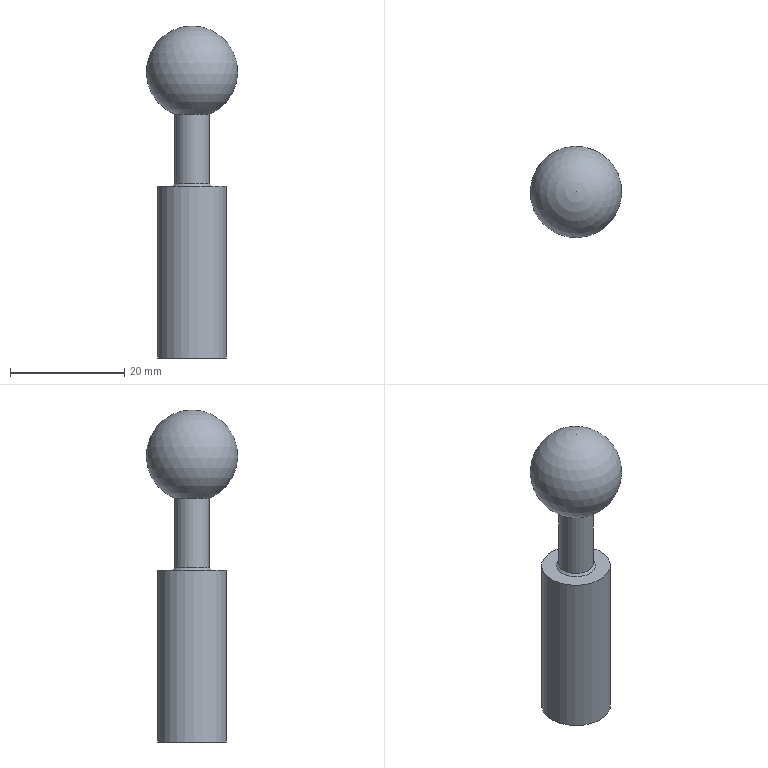Component | NX | GUIDE_POST | 1 solid | 6 faces | box 16 x 16 x 58 mm | volume 5887 mm3 | cylinder 2 | plane 2 | sphere 1 | cone 1 | commonest cylinder face diameters 6 x1 12 x1
STEP:
#1=CARTESIAN_POINT('',(0.,0.,0.));
#2=DIRECTION('',(0.,0.,1.));
#3=DIRECTION('',(1.,0.,0.));
#4=AXIS2_PLACEMENT_3D('',#1,#2,#3);
#5=CARTESIAN_POINT('',(-71.09,-2.544,40.4));
#6=VERTEX_POINT('',#5);
#7=CARTESIAN_POINT('',(-69.5,-0.,40.4));
#8=DIRECTION('',(0.,0.,1.));
#9=DIRECTION('',(-0.53,-0.848,0.));
#10=AXIS2_PLACEMENT_3D('',#7,#8,#9);
#11=CIRCLE('',#10,3.);
#12=CARTESIAN_POINT('',(-69.5,-0.,10.));
#13=DIRECTION('',(0.,0.,-1.));
#14=DIRECTION('',(-0.53,-0.848,0.));
#15=AXIS2_PLACEMENT_3D('',#12,#13,#14);
#16=CYLINDRICAL_SURFACE('',#15,3.);
#17=CARTESIAN_POINT('',(6.283,-30.4));
#18=DIRECTION('',(-1.,0.));
#19=VECTOR('',#18,1.);
#20=LINE('',#17,#19);
#21=(GEOMETRIC_REPRESENTATION_CONTEXT(2)PARAMETRIC_REPRESENTATION_CONTEXT()REPRESENTATION_CONTEXT('',''));
#22=DEFINITIONAL_REPRESENTATION('',(#20),#21);
#23=PCURVE('',#16,#22);
#24=CARTESIAN_POINT('',(-69.5,-0.,40.));
#25=DIRECTION('',(0.,0.,-1.));
#26=DIRECTION('',(-0.53,-0.848,0.));
#27=AXIS2_PLACEMENT_3D('',#24,#25,#26);
#28=CONICAL_SURFACE('',#27,3.4,0.7854);
#29=CARTESIAN_POINT('',(6.283,-0.4));
#30=DIRECTION('',(-1.,0.));
#31=VECTOR('',#30,1.);
#32=LINE('',#29,#31);
#33=(GEOMETRIC_REPRESENTATION_CONTEXT(2)PARAMETRIC_REPRESENTATION_CONTEXT()REPRESENTATION_CONTEXT('',''));
#34=DEFINITIONAL_REPRESENTATION('',(#32),#33);
#35=PCURVE('',#28,#34);
#36=SURFACE_CURVE('',#11,(#23,#35),.PCURVE_S1.);
#37=EDGE_CURVE('',#6,#6,#36,.T.);
#38=ORIENTED_EDGE('',*,*,#37,.T.);
#39=CARTESIAN_POINT('',(-71.09,-2.544,52.584));
#40=VERTEX_POINT('',#39);
#41=CARTESIAN_POINT('',(-71.09,-2.544,52.584));
#42=CARTESIAN_POINT('',(-71.09,-2.544,40.4));
#43=B_SPLINE_CURVE_WITH_KNOTS('',1,(#41,#42),.UNSPECIFIED.,.F.,.F.,(2,2),(-42.584,-30.4),.PIECEWISE_BEZIER_KNOTS.);
#44=CARTESIAN_POINT('',(0.,0.));
#45=DIRECTION('',(0.,1.));
#46=VECTOR('',#45,1.);
#47=LINE('',#44,#46);
#48=(GEOMETRIC_REPRESENTATION_CONTEXT(2)PARAMETRIC_REPRESENTATION_CONTEXT()REPRESENTATION_CONTEXT('',''));
#49=DEFINITIONAL_REPRESENTATION('',(#47),#48);
#50=PCURVE('',#16,#49);
#51=CARTESIAN_POINT('',(6.283,0.));
#52=DIRECTION('',(0.,1.));
#53=VECTOR('',#52,1.);
#54=LINE('',#51,#53);
#55=(GEOMETRIC_REPRESENTATION_CONTEXT(2)PARAMETRIC_REPRESENTATION_CONTEXT()REPRESENTATION_CONTEXT('',''));
#56=DEFINITIONAL_REPRESENTATION('',(#54),#55);
#57=PCURVE('',#16,#56);
#58=SEAM_CURVE('',#43,(#50,#57),.PCURVE_S1.);
#59=EDGE_CURVE('',#40,#6,#58,.T.);
#60=ORIENTED_EDGE('',*,*,#59,.F.);
#61=CARTESIAN_POINT('',(-67.91,2.544,52.584));
#62=VERTEX_POINT('',#61);
#63=CARTESIAN_POINT('',(-69.5,-0.,52.584));
#64=DIRECTION('',(0.,0.,-1.));
#65=DIRECTION('',(0.53,0.848,0.));
#66=AXIS2_PLACEMENT_3D('',#63,#64,#65);
#67=CIRCLE('',#66,3.);
#68=CARTESIAN_POINT('',(-3.142,-42.584));
#69=DIRECTION('',(1.,0.));
#70=VECTOR('',#69,1.);
#71=LINE('',#68,#70);
#72=(GEOMETRIC_REPRESENTATION_CONTEXT(2)PARAMETRIC_REPRESENTATION_CONTEXT()REPRESENTATION_CONTEXT('',''));
#73=DEFINITIONAL_REPRESENTATION('',(#71),#72);
#74=PCURVE('',#16,#73);
#75=CARTESIAN_POINT('',(-69.5,-0.,60.));
#76=DIRECTION('',(0.,0.,1.));
#77=DIRECTION('',(0.53,0.848,-0.));
#78=AXIS2_PLACEMENT_3D('',#75,#76,#77);
#79=SPHERICAL_SURFACE('',#78,8.);
#80=CARTESIAN_POINT('',(3.142,-1.186));
#81=CARTESIAN_POINT('',(3.094,-1.186));
#82=CARTESIAN_POINT('',(2.999,-1.186));
#83=CARTESIAN_POINT('',(2.856,-1.186));
#84=CARTESIAN_POINT('',(2.713,-1.186));
#85=CARTESIAN_POINT('',(2.57,-1.186));
#86=CARTESIAN_POINT('',(2.428,-1.186));
#87=CARTESIAN_POINT('',(2.285,-1.186));
#88=CARTESIAN_POINT('',(2.142,-1.186));
#89=CARTESIAN_POINT('',(1.999,-1.186));
#90=CARTESIAN_POINT('',(1.856,-1.186));
#91=CARTESIAN_POINT('',(1.714,-1.186));
#92=CARTESIAN_POINT('',(1.571,-1.186));
#93=CARTESIAN_POINT('',(1.428,-1.186));
#94=CARTESIAN_POINT('',(1.285,-1.186));
#95=CARTESIAN_POINT('',(1.142,-1.186));
#96=CARTESIAN_POINT('',(0.9996,-1.186));
#97=CARTESIAN_POINT('',(0.8568,-1.186));
#98=CARTESIAN_POINT('',(0.714,-1.186));
#99=CARTESIAN_POINT('',(0.5712,-1.186));
#100=CARTESIAN_POINT('',(0.4284,-1.186));
#101=CARTESIAN_POINT('',(0.2856,-1.186));
#102=CARTESIAN_POINT('',(0.1428,-1.186));
#103=CARTESIAN_POINT('',(0.0476,-1.186));
#104=CARTESIAN_POINT('',(0.,-1.186));
#105=B_SPLINE_CURVE_WITH_KNOTS('',3,(#80,#81,#82,#83,#84,#85,#86,#87,#88,#89,#90,#91,#92,#93,#94,#95,#96,#97,#98,#99,#100,#101,#102,#103,#104),.UNSPECIFIED.,.F.,.F.,(4,1,1,1,1,1,1,1,1,1,1,1,1,1,1,1,1,1,1,1,1,1,4),(3.142,3.284,3.427,3.57,3.713,3.856,3.998,4.141,4.284,4.427,4.57,4.712,4.855,4.998,5.141,5.284,5.426,5.569,5.712,5.855,5.998,6.14,6.283),.QUASI_UNIFORM_KNOTS.);
#106=(GEOMETRIC_REPRESENTATION_CONTEXT(2)PARAMETRIC_REPRESENTATION_CONTEXT()REPRESENTATION_CONTEXT('',''));
#107=DEFINITIONAL_REPRESENTATION('',(#105),#106);
#108=PCURVE('',#79,#107);
#109=SURFACE_CURVE('',#67,(#74,#108),.PCURVE_S1.);
#110=EDGE_CURVE('',#40,#62,#109,.T.);
#111=ORIENTED_EDGE('',*,*,#110,.T.);
#112=CARTESIAN_POINT('',(-69.5,-0.,52.584));
#113=DIRECTION('',(0.,0.,-1.));
#114=DIRECTION('',(0.53,0.848,0.));
#115=AXIS2_PLACEMENT_3D('',#112,#113,#114);
#116=CIRCLE('',#115,3.);
#117=CARTESIAN_POINT('',(3.142,-42.584));
#118=DIRECTION('',(1.,0.));
#119=VECTOR('',#118,1.);
#120=LINE('',#117,#119);
#121=(GEOMETRIC_REPRESENTATION_CONTEXT(2)PARAMETRIC_REPRESENTATION_CONTEXT()REPRESENTATION_CONTEXT('',''));
#122=DEFINITIONAL_REPRESENTATION('',(#120),#121);
#123=PCURVE('',#16,#122);
#124=CARTESIAN_POINT('',(6.283,-1.186));
#125=CARTESIAN_POINT('',(6.236,-1.186));
#126=CARTESIAN_POINT('',(6.14,-1.186));
#127=CARTESIAN_POINT('',(5.998,-1.186));
#128=CARTESIAN_POINT('',(5.855,-1.186));
#129=CARTESIAN_POINT('',(5.712,-1.186));
#130=CARTESIAN_POINT('',(5.569,-1.186));
#131=CARTESIAN_POINT('',(5.426,-1.186));
#132=CARTESIAN_POINT('',(5.284,-1.186));
#133=CARTESIAN_POINT('',(5.141,-1.186));
#134=CARTESIAN_POINT('',(4.998,-1.186));
#135=CARTESIAN_POINT('',(4.855,-1.186));
#136=CARTESIAN_POINT('',(4.712,-1.186));
#137=CARTESIAN_POINT('',(4.57,-1.186));
#138=CARTESIAN_POINT('',(4.427,-1.186));
#139=CARTESIAN_POINT('',(4.284,-1.186));
#140=CARTESIAN_POINT('',(4.141,-1.186));
#141=CARTESIAN_POINT('',(3.998,-1.186));
#142=CARTESIAN_POINT('',(3.856,-1.186));
#143=CARTESIAN_POINT('',(3.713,-1.186));
#144=CARTESIAN_POINT('',(3.57,-1.186));
#145=CARTESIAN_POINT('',(3.427,-1.186));
#146=CARTESIAN_POINT('',(3.284,-1.186));
#147=CARTESIAN_POINT('',(3.189,-1.186));
#148=CARTESIAN_POINT('',(3.142,-1.186));
#149=B_SPLINE_CURVE_WITH_KNOTS('',3,(#124,#125,#126,#127,#128,#129,#130,#131,#132,#133,#134,#135,#136,#137,#138,#139,#140,#141,#142,#143,#144,#145,#146,#147,#148),.UNSPECIFIED.,.F.,.F.,(4,1,1,1,1,1,1,1,1,1,1,1,1,1,1,1,1,1,1,1,1,1,4),(0.,0.1428,0.2856,0.4284,0.5712,0.714,0.8568,0.9996,1.142,1.285,1.428,1.571,1.714,1.856,1.999,2.142,2.285,2.428,2.57,2.713,2.856,2.999,3.142),.QUASI_UNIFORM_KNOTS.);
#150=(GEOMETRIC_REPRESENTATION_CONTEXT(2)PARAMETRIC_REPRESENTATION_CONTEXT()REPRESENTATION_CONTEXT('',''));
#151=DEFINITIONAL_REPRESENTATION('',(#149),#150);
#152=PCURVE('',#79,#151);
#153=SURFACE_CURVE('',#116,(#123,#152),.PCURVE_S1.);
#154=EDGE_CURVE('',#62,#40,#153,.T.);
#155=ORIENTED_EDGE('',*,*,#154,.T.);
#156=ORIENTED_EDGE('',*,*,#59,.T.);
#157=EDGE_LOOP('',(#38,#60,#111,#155,#156));
#158=FACE_BOUND('',#157,.T.);
#159=ADVANCED_FACE('',(#158),#16,.T.);
#160=CARTESIAN_POINT('',(-71.302,-2.883,40.));
#161=VERTEX_POINT('',#160);
#162=CARTESIAN_POINT('',(-69.5,-0.,40.));
#163=DIRECTION('',(0.,0.,-1.));
#164=DIRECTION('',(-0.53,-0.848,0.));
#165=AXIS2_PLACEMENT_3D('',#162,#163,#164);
#166=CIRCLE('',#165,3.4);
#167=CARTESIAN_POINT('',(-72.044,1.59,40.));
#168=DIRECTION('',(0.,0.,-1.));
#169=DIRECTION('',(-0.53,-0.848,0.));
#170=AXIS2_PLACEMENT_3D('',#167,#168,#169);
#171=PLANE('',#170);
#172=CARTESIAN_POINT('',(-0.,-3.));
#173=DIRECTION('',(1.,0.));
#174=AXIS2_PLACEMENT_2D('',#172,#173);
#175=CIRCLE('',#174,3.4);
#176=(GEOMETRIC_REPRESENTATION_CONTEXT(2)PARAMETRIC_REPRESENTATION_CONTEXT()REPRESENTATION_CONTEXT('',''));
#177=DEFINITIONAL_REPRESENTATION('',(#175),#176);
#178=PCURVE('',#171,#177);
#179=CARTESIAN_POINT('',(0.,0.));
#180=DIRECTION('',(1.,0.));
#181=VECTOR('',#180,1.);
#182=LINE('',#179,#181);
#183=(GEOMETRIC_REPRESENTATION_CONTEXT(2)PARAMETRIC_REPRESENTATION_CONTEXT()REPRESENTATION_CONTEXT('',''));
#184=DEFINITIONAL_REPRESENTATION('',(#182),#183);
#185=PCURVE('',#28,#184);
#186=SURFACE_CURVE('',#166,(#178,#185),.PCURVE_S1.);
#187=EDGE_CURVE('',#161,#161,#186,.T.);
#188=ORIENTED_EDGE('',*,*,#187,.T.);
#189=EDGE_LOOP('',(#188));
#190=FACE_BOUND('',#189,.T.);
#191=CARTESIAN_POINT('',(-72.68,-5.088,40.));
#192=VERTEX_POINT('',#191);
#193=CARTESIAN_POINT('',(-69.5,-0.,40.));
#194=DIRECTION('',(0.,0.,-1.));
#195=DIRECTION('',(-0.53,-0.848,0.));
#196=AXIS2_PLACEMENT_3D('',#193,#194,#195);
#197=CIRCLE('',#196,6.);
#198=CARTESIAN_POINT('',(-0.,-3.));
#199=DIRECTION('',(1.,0.));
#200=AXIS2_PLACEMENT_2D('',#198,#199);
#201=CIRCLE('',#200,6.);
#202=(GEOMETRIC_REPRESENTATION_CONTEXT(2)PARAMETRIC_REPRESENTATION_CONTEXT()REPRESENTATION_CONTEXT('',''));
#203=DEFINITIONAL_REPRESENTATION('',(#201),#202);
#204=PCURVE('',#171,#203);
#205=CARTESIAN_POINT('',(-69.5,-0.,10.));
#206=DIRECTION('',(0.,0.,-1.));
#207=DIRECTION('',(-0.53,-0.848,0.));
#208=AXIS2_PLACEMENT_3D('',#205,#206,#207);
#209=CYLINDRICAL_SURFACE('',#208,6.);
#210=CARTESIAN_POINT('',(0.,-30.));
#211=DIRECTION('',(1.,0.));
#212=VECTOR('',#211,1.);
#213=LINE('',#210,#212);
#214=(GEOMETRIC_REPRESENTATION_CONTEXT(2)PARAMETRIC_REPRESENTATION_CONTEXT()REPRESENTATION_CONTEXT('',''));
#215=DEFINITIONAL_REPRESENTATION('',(#213),#214);
#216=PCURVE('',#209,#215);
#217=SURFACE_CURVE('',#197,(#204,#216),.PCURVE_S1.);
#218=EDGE_CURVE('',#192,#192,#217,.T.);
#219=ORIENTED_EDGE('',*,*,#218,.F.);
#220=EDGE_LOOP('',(#219));
#221=FACE_BOUND('',#220,.T.);
#222=ADVANCED_FACE('',(#190,#221),#171,.F.);
#223=CARTESIAN_POINT('',(-72.68,-5.088,10.));
#224=VERTEX_POINT('',#223);
#225=CARTESIAN_POINT('',(-69.5,-0.,10.));
#226=DIRECTION('',(0.,0.,-1.));
#227=DIRECTION('',(-0.53,-0.848,0.));
#228=AXIS2_PLACEMENT_3D('',#225,#226,#227);
#229=CIRCLE('',#228,6.);
#230=CARTESIAN_POINT('',(0.,0.));
#231=DIRECTION('',(1.,0.));
#232=VECTOR('',#231,1.);
#233=LINE('',#230,#232);
#234=(GEOMETRIC_REPRESENTATION_CONTEXT(2)PARAMETRIC_REPRESENTATION_CONTEXT()REPRESENTATION_CONTEXT('',''));
#235=DEFINITIONAL_REPRESENTATION('',(#233),#234);
#236=PCURVE('',#209,#235);
#237=CARTESIAN_POINT('',(-74.588,3.18,10.));
#238=DIRECTION('',(0.,0.,1.));
#239=DIRECTION('',(0.53,0.848,0.));
#240=AXIS2_PLACEMENT_3D('',#237,#238,#239);
#241=PLANE('',#240);
#242=CARTESIAN_POINT('',(-6.,-6.));
#243=CARTESIAN_POINT('',(-6.,4.392));
#244=CARTESIAN_POINT('',(3.,-0.8038));
#245=CARTESIAN_POINT('',(12.,-6.));
#246=CARTESIAN_POINT('',(3.,-11.196));
#247=CARTESIAN_POINT('',(-6.,-16.392));
#248=CARTESIAN_POINT('',(-6.,-6.));
#249=(BOUNDED_CURVE()B_SPLINE_CURVE(2,(#242,#243,#244,#245,#246,#247,#248),.UNSPECIFIED.,.T.,.F.)B_SPLINE_CURVE_WITH_KNOTS((1,2,2,2,2,1),(-2.094,0.,2.094,4.189,6.283,8.378),.UNSPECIFIED.)CURVE()GEOMETRIC_REPRESENTATION_ITEM()RATIONAL_B_SPLINE_CURVE((1.,0.5,1.,0.5,1.,0.5,1.))REPRESENTATION_ITEM(''));
#250=(GEOMETRIC_REPRESENTATION_CONTEXT(2)PARAMETRIC_REPRESENTATION_CONTEXT()REPRESENTATION_CONTEXT('',''));
#251=DEFINITIONAL_REPRESENTATION('',(#249),#250);
#252=PCURVE('',#241,#251);
#253=SURFACE_CURVE('',#229,(#236,#252),.PCURVE_S1.);
#254=EDGE_CURVE('',#224,#224,#253,.T.);
#255=ORIENTED_EDGE('',*,*,#254,.F.);
#256=CARTESIAN_POINT('',(-72.68,-5.088,40.));
#257=CARTESIAN_POINT('',(-72.68,-5.088,10.));
#258=B_SPLINE_CURVE_WITH_KNOTS('',1,(#256,#257),.UNSPECIFIED.,.F.,.F.,(2,2),(-30.,0.),.PIECEWISE_BEZIER_KNOTS.);
#259=CARTESIAN_POINT('',(0.,0.));
#260=DIRECTION('',(0.,1.));
#261=VECTOR('',#260,1.);
#262=LINE('',#259,#261);
#263=(GEOMETRIC_REPRESENTATION_CONTEXT(2)PARAMETRIC_REPRESENTATION_CONTEXT()REPRESENTATION_CONTEXT('',''));
#264=DEFINITIONAL_REPRESENTATION('',(#262),#263);
#265=PCURVE('',#209,#264);
#266=CARTESIAN_POINT('',(6.283,0.));
#267=DIRECTION('',(0.,1.));
#268=VECTOR('',#267,1.);
#269=LINE('',#266,#268);
#270=(GEOMETRIC_REPRESENTATION_CONTEXT(2)PARAMETRIC_REPRESENTATION_CONTEXT()REPRESENTATION_CONTEXT('',''));
#271=DEFINITIONAL_REPRESENTATION('',(#269),#270);
#272=PCURVE('',#209,#271);
#273=SEAM_CURVE('',#258,(#265,#272),.PCURVE_S1.);
#274=EDGE_CURVE('',#192,#224,#273,.T.);
#275=ORIENTED_EDGE('',*,*,#274,.F.);
#276=ORIENTED_EDGE('',*,*,#218,.T.);
#277=ORIENTED_EDGE('',*,*,#274,.T.);
#278=EDGE_LOOP('',(#255,#275,#276,#277));
#279=FACE_BOUND('',#278,.T.);
#280=ADVANCED_FACE('',(#279),#209,.T.);
#281=ORIENTED_EDGE('',*,*,#254,.T.);
#282=EDGE_LOOP('',(#281));
#283=FACE_BOUND('',#282,.T.);
#284=ADVANCED_FACE('',(#283),#241,.F.);
#285=ORIENTED_EDGE('',*,*,#154,.F.);
#286=CARTESIAN_POINT('',(-69.5,-0.,68.));
#287=VERTEX_POINT('',#286);
#288=CARTESIAN_POINT('',(-67.91,2.544,52.584));
#289=CARTESIAN_POINT('',(-66.555,4.711,53.618));
#290=CARTESIAN_POINT('',(-65.416,6.533,55.659));
#291=CARTESIAN_POINT('',(-64.738,7.618,58.518));
#292=CARTESIAN_POINT('',(-64.712,7.66,61.758));
#293=CARTESIAN_POINT('',(-65.38,6.591,64.742));
#294=CARTESIAN_POINT('',(-66.577,4.676,66.914));
#295=CARTESIAN_POINT('',(-68.039,2.338,68.));
#296=CARTESIAN_POINT('',(-69.5,-0.,68.));
#297=B_SPLINE_CURVE_WITH_KNOTS('',8,(#288,#289,#290,#291,#292,#293,#294,#295,#296),.UNSPECIFIED.,.F.,.F.,(9,9),(-1.186,1.571),.PIECEWISE_BEZIER_KNOTS.);
#298=CARTESIAN_POINT('',(6.283,0.));
#299=DIRECTION('',(0.,1.));
#300=VECTOR('',#299,1.);
#301=LINE('',#298,#300);
#302=(GEOMETRIC_REPRESENTATION_CONTEXT(2)PARAMETRIC_REPRESENTATION_CONTEXT()REPRESENTATION_CONTEXT('',''));
#303=DEFINITIONAL_REPRESENTATION('',(#301),#302);
#304=PCURVE('',#79,#303);
#305=CARTESIAN_POINT('',(0.,0.));
#306=DIRECTION('',(0.,1.));
#307=VECTOR('',#306,1.);
#308=LINE('',#305,#307);
#309=(GEOMETRIC_REPRESENTATION_CONTEXT(2)PARAMETRIC_REPRESENTATION_CONTEXT()REPRESENTATION_CONTEXT('',''));
#310=DEFINITIONAL_REPRESENTATION('',(#308),#309);
#311=PCURVE('',#79,#310);
#312=SEAM_CURVE('',#297,(#304,#311),.PCURVE_S1.);
#313=EDGE_CURVE('',#62,#287,#312,.T.);
#314=ORIENTED_EDGE('',*,*,#313,.T.);
#315=ORIENTED_EDGE('',*,*,#313,.F.);
#316=ORIENTED_EDGE('',*,*,#110,.F.);
#317=EDGE_LOOP('',(#285,#314,#315,#316));
#318=FACE_BOUND('',#317,.T.);
#319=ADVANCED_FACE('',(#318),#79,.T.);
#320=ORIENTED_EDGE('',*,*,#37,.F.);
#321=CARTESIAN_POINT('',(-71.09,-2.544,40.4));
#322=CARTESIAN_POINT('',(-71.302,-2.883,40.));
#323=B_SPLINE_CURVE_WITH_KNOTS('',1,(#321,#322),.UNSPECIFIED.,.F.,.F.,(2,2),(-0.5657,0.),.PIECEWISE_BEZIER_KNOTS.);
#324=CARTESIAN_POINT('',(6.283,0.));
#325=DIRECTION('',(0.,1.));
#326=VECTOR('',#325,1.);
#327=LINE('',#324,#326);
#328=(GEOMETRIC_REPRESENTATION_CONTEXT(2)PARAMETRIC_REPRESENTATION_CONTEXT()REPRESENTATION_CONTEXT('',''));
#329=DEFINITIONAL_REPRESENTATION('',(#327),#328);
#330=PCURVE('',#28,#329);
#331=CARTESIAN_POINT('',(0.,0.));
#332=DIRECTION('',(0.,1.));
#333=VECTOR('',#332,1.);
#334=LINE('',#331,#333);
#335=(GEOMETRIC_REPRESENTATION_CONTEXT(2)PARAMETRIC_REPRESENTATION_CONTEXT()REPRESENTATION_CONTEXT('',''));
#336=DEFINITIONAL_REPRESENTATION('',(#334),#335);
#337=PCURVE('',#28,#336);
#338=SEAM_CURVE('',#323,(#330,#337),.PCURVE_S1.);
#339=EDGE_CURVE('',#6,#161,#338,.T.);
#340=ORIENTED_EDGE('',*,*,#339,.T.);
#341=ORIENTED_EDGE('',*,*,#187,.F.);
#342=ORIENTED_EDGE('',*,*,#339,.F.);
#343=EDGE_LOOP('',(#320,#340,#341,#342));
#344=FACE_BOUND('',#343,.T.);
#345=ADVANCED_FACE('',(#344),#28,.T.);
#346=CLOSED_SHELL('',(#159,#222,#280,#284,#319,#345));
#347=MANIFOLD_SOLID_BREP('',#346);
#348=(LENGTH_UNIT()NAMED_UNIT(*)SI_UNIT(.MILLI.,.METRE.));
#349=UNCERTAINTY_MEASURE_WITH_UNIT(LENGTH_MEASURE(0.00001),#348,'','');
#350=(NAMED_UNIT(*)PLANE_ANGLE_UNIT()SI_UNIT($,.RADIAN.));
#351=(NAMED_UNIT(*)SI_UNIT($,.STERADIAN.)SOLID_ANGLE_UNIT());
#352=(GEOMETRIC_REPRESENTATION_CONTEXT(3)GLOBAL_UNCERTAINTY_ASSIGNED_CONTEXT((#349))GLOBAL_UNIT_ASSIGNED_CONTEXT((#348,#350,#351))REPRESENTATION_CONTEXT('',''));
#353=ADVANCED_BREP_SHAPE_REPRESENTATION('',(#4,#347),#352);